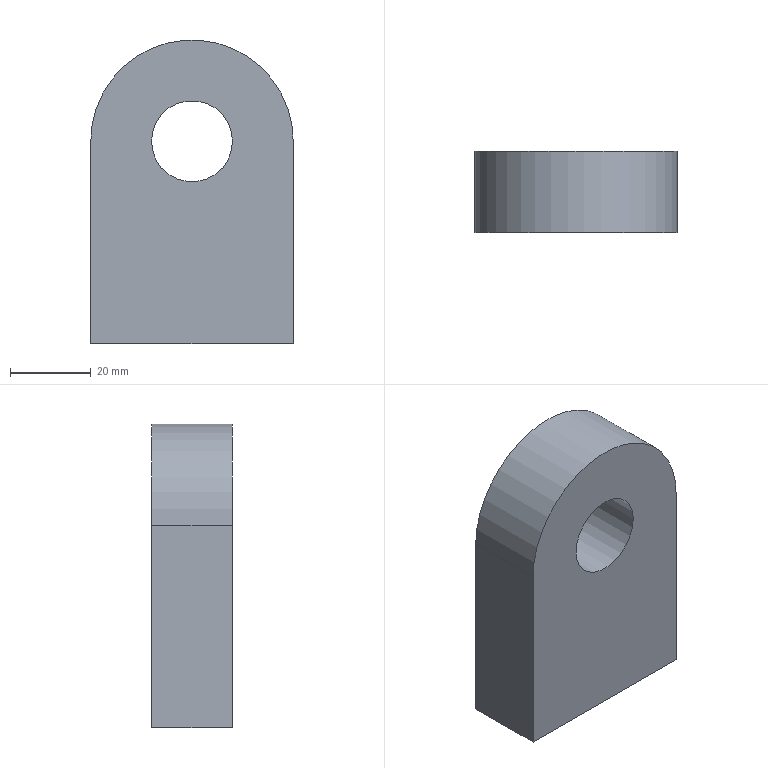Component | NX | BRACKET_1 | 1 solid | 13 faces | box 50 x 20 x 75 mm | volume 62277 mm3 | plane 5 | cylinder 4 | cone 4 | commonest cylinder face diameters 6.8 x2 50 x1 20 x1
STEP:
#1=CARTESIAN_POINT('',(0.,0.,0.));
#2=DIRECTION('',(0.,0.,1.));
#3=DIRECTION('',(1.,0.,0.));
#4=AXIS2_PLACEMENT_3D('',#1,#2,#3);
#5=CARTESIAN_POINT('',(40.5,45.,62.));
#6=VERTEX_POINT('',#5);
#7=CARTESIAN_POINT('',(40.5,45.,12.));
#8=VERTEX_POINT('',#7);
#9=CARTESIAN_POINT('',(40.5,45.,62.));
#10=DIRECTION('',(-0.,0.,-1.));
#11=VECTOR('',#10,1.);
#12=LINE('',#9,#11);
#13=CARTESIAN_POINT('',(40.5,25.,62.));
#14=DIRECTION('',(1.,0.,-0.));
#15=DIRECTION('',(0.,0.,1.));
#16=AXIS2_PLACEMENT_3D('',#13,#14,#15);
#17=PLANE('',#16);
#18=CARTESIAN_POINT('',(0.,-20.));
#19=DIRECTION('',(-1.,0.));
#20=VECTOR('',#19,1.);
#21=LINE('',#18,#20);
#22=(GEOMETRIC_REPRESENTATION_CONTEXT(2)PARAMETRIC_REPRESENTATION_CONTEXT()REPRESENTATION_CONTEXT('',''));
#23=DEFINITIONAL_REPRESENTATION('',(#21),#22);
#24=PCURVE('',#17,#23);
#25=CARTESIAN_POINT('',(65.5,45.,62.));
#26=DIRECTION('',(0.,-1.,0.));
#27=DIRECTION('',(0.,0.,-1.));
#28=AXIS2_PLACEMENT_3D('',#25,#26,#27);
#29=PLANE('',#28);
#30=CARTESIAN_POINT('',(0.,-25.));
#31=DIRECTION('',(1.,-0.));
#32=VECTOR('',#31,1.);
#33=LINE('',#30,#32);
#34=(GEOMETRIC_REPRESENTATION_CONTEXT(2)PARAMETRIC_REPRESENTATION_CONTEXT()REPRESENTATION_CONTEXT('',''));
#35=DEFINITIONAL_REPRESENTATION('',(#33),#34);
#36=PCURVE('',#29,#35);
#37=SURFACE_CURVE('',#12,(#24,#36),.PCURVE_S1.);
#38=EDGE_CURVE('',#6,#8,#37,.T.);
#39=ORIENTED_EDGE('',*,*,#38,.T.);
#40=CARTESIAN_POINT('',(40.5,25.,12.));
#41=VERTEX_POINT('',#40);
#42=CARTESIAN_POINT('',(40.5,25.,12.));
#43=DIRECTION('',(0.,1.,0.));
#44=VECTOR('',#43,1.);
#45=LINE('',#42,#44);
#46=CARTESIAN_POINT('',(-50.,0.));
#47=DIRECTION('',(0.,-1.));
#48=VECTOR('',#47,1.);
#49=LINE('',#46,#48);
#50=(GEOMETRIC_REPRESENTATION_CONTEXT(2)PARAMETRIC_REPRESENTATION_CONTEXT()REPRESENTATION_CONTEXT('',''));
#51=DEFINITIONAL_REPRESENTATION('',(#49),#50);
#52=PCURVE('',#17,#51);
#53=CARTESIAN_POINT('',(40.5,25.,12.));
#54=DIRECTION('',(-0.,0.,1.));
#55=DIRECTION('',(-1.,0.,-0.));
#56=AXIS2_PLACEMENT_3D('',#53,#54,#55);
#57=PLANE('',#56);
#58=CARTESIAN_POINT('',(0.,0.));
#59=DIRECTION('',(0.,-1.));
#60=VECTOR('',#59,1.);
#61=LINE('',#58,#60);
#62=(GEOMETRIC_REPRESENTATION_CONTEXT(2)PARAMETRIC_REPRESENTATION_CONTEXT()REPRESENTATION_CONTEXT('',''));
#63=DEFINITIONAL_REPRESENTATION('',(#61),#62);
#64=PCURVE('',#57,#63);
#65=SURFACE_CURVE('',#45,(#52,#64),.PCURVE_S1.);
#66=EDGE_CURVE('',#41,#8,#65,.T.);
#67=ORIENTED_EDGE('',*,*,#66,.F.);
#68=CARTESIAN_POINT('',(40.5,25.,62.));
#69=VERTEX_POINT('',#68);
#70=CARTESIAN_POINT('',(40.5,25.,62.));
#71=DIRECTION('',(-0.,0.,-1.));
#72=VECTOR('',#71,1.);
#73=LINE('',#70,#72);
#74=CARTESIAN_POINT('',(0.,0.));
#75=DIRECTION('',(-1.,0.));
#76=VECTOR('',#75,1.);
#77=LINE('',#74,#76);
#78=(GEOMETRIC_REPRESENTATION_CONTEXT(2)PARAMETRIC_REPRESENTATION_CONTEXT()REPRESENTATION_CONTEXT('',''));
#79=DEFINITIONAL_REPRESENTATION('',(#77),#78);
#80=PCURVE('',#17,#79);
#81=CARTESIAN_POINT('',(65.5,25.,62.));
#82=DIRECTION('',(0.,-1.,0.));
#83=DIRECTION('',(0.,0.,-1.));
#84=AXIS2_PLACEMENT_3D('',#81,#82,#83);
#85=PLANE('',#84);
#86=CARTESIAN_POINT('',(0.,-25.));
#87=DIRECTION('',(1.,-0.));
#88=VECTOR('',#87,1.);
#89=LINE('',#86,#88);
#90=(GEOMETRIC_REPRESENTATION_CONTEXT(2)PARAMETRIC_REPRESENTATION_CONTEXT()REPRESENTATION_CONTEXT('',''));
#91=DEFINITIONAL_REPRESENTATION('',(#89),#90);
#92=PCURVE('',#85,#91);
#93=SURFACE_CURVE('',#73,(#80,#92),.PCURVE_S1.);
#94=EDGE_CURVE('',#69,#41,#93,.T.);
#95=ORIENTED_EDGE('',*,*,#94,.F.);
#96=CARTESIAN_POINT('',(40.5,25.,62.));
#97=DIRECTION('',(0.,1.,0.));
#98=VECTOR('',#97,1.);
#99=LINE('',#96,#98);
#100=CARTESIAN_POINT('',(0.,0.));
#101=DIRECTION('',(0.,-1.));
#102=VECTOR('',#101,1.);
#103=LINE('',#100,#102);
#104=(GEOMETRIC_REPRESENTATION_CONTEXT(2)PARAMETRIC_REPRESENTATION_CONTEXT()REPRESENTATION_CONTEXT('',''));
#105=DEFINITIONAL_REPRESENTATION('',(#103),#104);
#106=PCURVE('',#17,#105);
#107=CARTESIAN_POINT('',(65.5,25.,62.));
#108=DIRECTION('',(0.,1.,0.));
#109=DIRECTION('',(0.,0.,1.));
#110=AXIS2_PLACEMENT_3D('',#107,#108,#109);
#111=CYLINDRICAL_SURFACE('',#110,25.);
#112=CARTESIAN_POINT('',(-1.571,0.));
#113=DIRECTION('',(0.,1.));
#114=VECTOR('',#113,1.);
#115=LINE('',#112,#114);
#116=(GEOMETRIC_REPRESENTATION_CONTEXT(2)PARAMETRIC_REPRESENTATION_CONTEXT()REPRESENTATION_CONTEXT('',''));
#117=DEFINITIONAL_REPRESENTATION('',(#115),#116);
#118=PCURVE('',#111,#117);
#119=SURFACE_CURVE('',#99,(#106,#118),.PCURVE_S1.);
#120=EDGE_CURVE('',#69,#6,#119,.T.);
#121=ORIENTED_EDGE('',*,*,#120,.T.);
#122=EDGE_LOOP('',(#39,#67,#95,#121));
#123=FACE_BOUND('',#122,.T.);
#124=ADVANCED_FACE('',(#123),#17,.F.);
#125=CARTESIAN_POINT('',(78.5,35.,12.));
#126=VERTEX_POINT('',#125);
#127=CARTESIAN_POINT('',(82.5,35.,12.));
#128=DIRECTION('',(-0.,0.,1.));
#129=DIRECTION('',(-1.,0.,-0.));
#130=AXIS2_PLACEMENT_3D('',#127,#128,#129);
#131=CIRCLE('',#130,4.);
#132=CARTESIAN_POINT('',(-42.,-10.));
#133=DIRECTION('',(1.,0.));
#134=AXIS2_PLACEMENT_2D('',#132,#133);
#135=CIRCLE('',#134,4.);
#136=(GEOMETRIC_REPRESENTATION_CONTEXT(2)PARAMETRIC_REPRESENTATION_CONTEXT()REPRESENTATION_CONTEXT('',''));
#137=DEFINITIONAL_REPRESENTATION('',(#135),#136);
#138=PCURVE('',#57,#137);
#139=CARTESIAN_POINT('',(82.5,35.,12.));
#140=DIRECTION('',(0.,0.,-1.));
#141=DIRECTION('',(0.,1.,0.));
#142=AXIS2_PLACEMENT_3D('',#139,#140,#141);
#143=CONICAL_SURFACE('',#142,4.,0.7854);
#144=CARTESIAN_POINT('',(10.996,0.));
#145=DIRECTION('',(-1.,0.));
#146=VECTOR('',#145,1.);
#147=LINE('',#144,#146);
#148=(GEOMETRIC_REPRESENTATION_CONTEXT(2)PARAMETRIC_REPRESENTATION_CONTEXT()REPRESENTATION_CONTEXT('',''));
#149=DEFINITIONAL_REPRESENTATION('',(#147),#148);
#150=PCURVE('',#143,#149);
#151=SURFACE_CURVE('',#131,(#138,#150),.PCURVE_S1.);
#152=EDGE_CURVE('',#126,#126,#151,.T.);
#153=ORIENTED_EDGE('',*,*,#152,.T.);
#154=EDGE_LOOP('',(#153));
#155=FACE_BOUND('',#154,.T.);
#156=CARTESIAN_POINT('',(44.5,35.,12.));
#157=VERTEX_POINT('',#156);
#158=CARTESIAN_POINT('',(48.5,35.,12.));
#159=DIRECTION('',(-0.,0.,1.));
#160=DIRECTION('',(-1.,0.,-0.));
#161=AXIS2_PLACEMENT_3D('',#158,#159,#160);
#162=CIRCLE('',#161,4.);
#163=CARTESIAN_POINT('',(-8.,-10.));
#164=DIRECTION('',(1.,0.));
#165=AXIS2_PLACEMENT_2D('',#163,#164);
#166=CIRCLE('',#165,4.);
#167=(GEOMETRIC_REPRESENTATION_CONTEXT(2)PARAMETRIC_REPRESENTATION_CONTEXT()REPRESENTATION_CONTEXT('',''));
#168=DEFINITIONAL_REPRESENTATION('',(#166),#167);
#169=PCURVE('',#57,#168);
#170=CARTESIAN_POINT('',(48.5,35.,12.));
#171=DIRECTION('',(0.,0.,-1.));
#172=DIRECTION('',(0.,1.,0.));
#173=AXIS2_PLACEMENT_3D('',#170,#171,#172);
#174=CONICAL_SURFACE('',#173,4.,0.7854);
#175=CARTESIAN_POINT('',(10.996,0.));
#176=DIRECTION('',(-1.,0.));
#177=VECTOR('',#176,1.);
#178=LINE('',#175,#177);
#179=(GEOMETRIC_REPRESENTATION_CONTEXT(2)PARAMETRIC_REPRESENTATION_CONTEXT()REPRESENTATION_CONTEXT('',''));
#180=DEFINITIONAL_REPRESENTATION('',(#178),#179);
#181=PCURVE('',#174,#180);
#182=SURFACE_CURVE('',#162,(#169,#181),.PCURVE_S1.);
#183=EDGE_CURVE('',#157,#157,#182,.T.);
#184=ORIENTED_EDGE('',*,*,#183,.T.);
#185=EDGE_LOOP('',(#184));
#186=FACE_BOUND('',#185,.T.);
#187=CARTESIAN_POINT('',(90.5,45.,12.));
#188=VERTEX_POINT('',#187);
#189=CARTESIAN_POINT('',(40.5,45.,12.));
#190=DIRECTION('',(1.,0.,0.));
#191=VECTOR('',#190,1.);
#192=LINE('',#189,#191);
#193=CARTESIAN_POINT('',(0.,-20.));
#194=DIRECTION('',(-1.,0.));
#195=VECTOR('',#194,1.);
#196=LINE('',#193,#195);
#197=(GEOMETRIC_REPRESENTATION_CONTEXT(2)PARAMETRIC_REPRESENTATION_CONTEXT()REPRESENTATION_CONTEXT('',''));
#198=DEFINITIONAL_REPRESENTATION('',(#196),#197);
#199=PCURVE('',#57,#198);
#200=CARTESIAN_POINT('',(50.,-25.));
#201=DIRECTION('',(-0.,1.));
#202=VECTOR('',#201,1.);
#203=LINE('',#200,#202);
#204=(GEOMETRIC_REPRESENTATION_CONTEXT(2)PARAMETRIC_REPRESENTATION_CONTEXT()REPRESENTATION_CONTEXT('',''));
#205=DEFINITIONAL_REPRESENTATION('',(#203),#204);
#206=PCURVE('',#29,#205);
#207=SURFACE_CURVE('',#192,(#199,#206),.PCURVE_S1.);
#208=EDGE_CURVE('',#8,#188,#207,.T.);
#209=ORIENTED_EDGE('',*,*,#208,.T.);
#210=CARTESIAN_POINT('',(90.5,25.,12.));
#211=VERTEX_POINT('',#210);
#212=CARTESIAN_POINT('',(90.5,25.,12.));
#213=DIRECTION('',(0.,1.,0.));
#214=VECTOR('',#213,1.);
#215=LINE('',#212,#214);
#216=CARTESIAN_POINT('',(-50.,0.));
#217=DIRECTION('',(0.,-1.));
#218=VECTOR('',#217,1.);
#219=LINE('',#216,#218);
#220=(GEOMETRIC_REPRESENTATION_CONTEXT(2)PARAMETRIC_REPRESENTATION_CONTEXT()REPRESENTATION_CONTEXT('',''));
#221=DEFINITIONAL_REPRESENTATION('',(#219),#220);
#222=PCURVE('',#57,#221);
#223=CARTESIAN_POINT('',(90.5,25.,12.));
#224=DIRECTION('',(-1.,0.,-0.));
#225=DIRECTION('',(0.,0.,-1.));
#226=AXIS2_PLACEMENT_3D('',#223,#224,#225);
#227=PLANE('',#226);
#228=CARTESIAN_POINT('',(0.,0.));
#229=DIRECTION('',(0.,-1.));
#230=VECTOR('',#229,1.);
#231=LINE('',#228,#230);
#232=(GEOMETRIC_REPRESENTATION_CONTEXT(2)PARAMETRIC_REPRESENTATION_CONTEXT()REPRESENTATION_CONTEXT('',''));
#233=DEFINITIONAL_REPRESENTATION('',(#231),#232);
#234=PCURVE('',#227,#233);
#235=SURFACE_CURVE('',#215,(#222,#234),.PCURVE_S1.);
#236=EDGE_CURVE('',#211,#188,#235,.T.);
#237=ORIENTED_EDGE('',*,*,#236,.F.);
#238=CARTESIAN_POINT('',(40.5,25.,12.));
#239=DIRECTION('',(1.,0.,0.));
#240=VECTOR('',#239,1.);
#241=LINE('',#238,#240);
#242=CARTESIAN_POINT('',(0.,0.));
#243=DIRECTION('',(-1.,0.));
#244=VECTOR('',#243,1.);
#245=LINE('',#242,#244);
#246=(GEOMETRIC_REPRESENTATION_CONTEXT(2)PARAMETRIC_REPRESENTATION_CONTEXT()REPRESENTATION_CONTEXT('',''));
#247=DEFINITIONAL_REPRESENTATION('',(#245),#246);
#248=PCURVE('',#57,#247);
#249=CARTESIAN_POINT('',(50.,-25.));
#250=DIRECTION('',(-0.,1.));
#251=VECTOR('',#250,1.);
#252=LINE('',#249,#251);
#253=(GEOMETRIC_REPRESENTATION_CONTEXT(2)PARAMETRIC_REPRESENTATION_CONTEXT()REPRESENTATION_CONTEXT('',''));
#254=DEFINITIONAL_REPRESENTATION('',(#252),#253);
#255=PCURVE('',#85,#254);
#256=SURFACE_CURVE('',#241,(#248,#255),.PCURVE_S1.);
#257=EDGE_CURVE('',#41,#211,#256,.T.);
#258=ORIENTED_EDGE('',*,*,#257,.F.);
#259=ORIENTED_EDGE('',*,*,#66,.T.);
#260=EDGE_LOOP('',(#209,#237,#258,#259));
#261=FACE_BOUND('',#260,.T.);
#262=ADVANCED_FACE('',(#155,#186,#261),#57,.F.);
#263=CARTESIAN_POINT('',(90.5,45.,62.));
#264=VERTEX_POINT('',#263);
#265=CARTESIAN_POINT('',(90.5,45.,12.));
#266=DIRECTION('',(-0.,0.,1.));
#267=VECTOR('',#266,1.);
#268=LINE('',#265,#267);
#269=CARTESIAN_POINT('',(0.,-20.));
#270=DIRECTION('',(-1.,0.));
#271=VECTOR('',#270,1.);
#272=LINE('',#269,#271);
#273=(GEOMETRIC_REPRESENTATION_CONTEXT(2)PARAMETRIC_REPRESENTATION_CONTEXT()REPRESENTATION_CONTEXT('',''));
#274=DEFINITIONAL_REPRESENTATION('',(#272),#273);
#275=PCURVE('',#227,#274);
#276=CARTESIAN_POINT('',(50.,25.));
#277=DIRECTION('',(-1.,-0.));
#278=VECTOR('',#277,1.);
#279=LINE('',#276,#278);
#280=(GEOMETRIC_REPRESENTATION_CONTEXT(2)PARAMETRIC_REPRESENTATION_CONTEXT()REPRESENTATION_CONTEXT('',''));
#281=DEFINITIONAL_REPRESENTATION('',(#279),#280);
#282=PCURVE('',#29,#281);
#283=SURFACE_CURVE('',#268,(#275,#282),.PCURVE_S1.);
#284=EDGE_CURVE('',#188,#264,#283,.T.);
#285=ORIENTED_EDGE('',*,*,#284,.T.);
#286=CARTESIAN_POINT('',(90.5,25.,62.));
#287=VERTEX_POINT('',#286);
#288=CARTESIAN_POINT('',(90.5,25.,62.));
#289=DIRECTION('',(0.,1.,0.));
#290=VECTOR('',#289,1.);
#291=LINE('',#288,#290);
#292=CARTESIAN_POINT('',(-50.,0.));
#293=DIRECTION('',(0.,-1.));
#294=VECTOR('',#293,1.);
#295=LINE('',#292,#294);
#296=(GEOMETRIC_REPRESENTATION_CONTEXT(2)PARAMETRIC_REPRESENTATION_CONTEXT()REPRESENTATION_CONTEXT('',''));
#297=DEFINITIONAL_REPRESENTATION('',(#295),#296);
#298=PCURVE('',#227,#297);
#299=CARTESIAN_POINT('',(1.571,0.));
#300=DIRECTION('',(0.,1.));
#301=VECTOR('',#300,1.);
#302=LINE('',#299,#301);
#303=(GEOMETRIC_REPRESENTATION_CONTEXT(2)PARAMETRIC_REPRESENTATION_CONTEXT()REPRESENTATION_CONTEXT('',''));
#304=DEFINITIONAL_REPRESENTATION('',(#302),#303);
#305=PCURVE('',#111,#304);
#306=SURFACE_CURVE('',#291,(#298,#305),.PCURVE_S1.);
#307=EDGE_CURVE('',#287,#264,#306,.T.);
#308=ORIENTED_EDGE('',*,*,#307,.F.);
#309=CARTESIAN_POINT('',(90.5,25.,12.));
#310=DIRECTION('',(-0.,0.,1.));
#311=VECTOR('',#310,1.);
#312=LINE('',#309,#311);
#313=CARTESIAN_POINT('',(0.,0.));
#314=DIRECTION('',(-1.,0.));
#315=VECTOR('',#314,1.);
#316=LINE('',#313,#315);
#317=(GEOMETRIC_REPRESENTATION_CONTEXT(2)PARAMETRIC_REPRESENTATION_CONTEXT()REPRESENTATION_CONTEXT('',''));
#318=DEFINITIONAL_REPRESENTATION('',(#316),#317);
#319=PCURVE('',#227,#318);
#320=CARTESIAN_POINT('',(50.,25.));
#321=DIRECTION('',(-1.,-0.));
#322=VECTOR('',#321,1.);
#323=LINE('',#320,#322);
#324=(GEOMETRIC_REPRESENTATION_CONTEXT(2)PARAMETRIC_REPRESENTATION_CONTEXT()REPRESENTATION_CONTEXT('',''));
#325=DEFINITIONAL_REPRESENTATION('',(#323),#324);
#326=PCURVE('',#85,#325);
#327=SURFACE_CURVE('',#312,(#319,#326),.PCURVE_S1.);
#328=EDGE_CURVE('',#211,#287,#327,.T.);
#329=ORIENTED_EDGE('',*,*,#328,.F.);
#330=ORIENTED_EDGE('',*,*,#236,.T.);
#331=EDGE_LOOP('',(#285,#308,#329,#330));
#332=FACE_BOUND('',#331,.T.);
#333=ADVANCED_FACE('',(#332),#227,.F.);
#334=CARTESIAN_POINT('',(65.5,45.,62.));
#335=DIRECTION('',(0.,-1.,0.));
#336=DIRECTION('',(1.,0.,0.));
#337=AXIS2_PLACEMENT_3D('',#334,#335,#336);
#338=CIRCLE('',#337,25.);
#339=CARTESIAN_POINT('',(1.571,20.));
#340=DIRECTION('',(-1.,0.));
#341=VECTOR('',#340,1.);
#342=LINE('',#339,#341);
#343=(GEOMETRIC_REPRESENTATION_CONTEXT(2)PARAMETRIC_REPRESENTATION_CONTEXT()REPRESENTATION_CONTEXT('',''));
#344=DEFINITIONAL_REPRESENTATION('',(#342),#343);
#345=PCURVE('',#111,#344);
#346=CARTESIAN_POINT('',(0.,0.));
#347=DIRECTION('',(0.,1.));
#348=AXIS2_PLACEMENT_2D('',#346,#347);
#349=CIRCLE('',#348,25.);
#350=(GEOMETRIC_REPRESENTATION_CONTEXT(2)PARAMETRIC_REPRESENTATION_CONTEXT()REPRESENTATION_CONTEXT('',''));
#351=DEFINITIONAL_REPRESENTATION('',(#349),#350);
#352=PCURVE('',#29,#351);
#353=SURFACE_CURVE('',#338,(#345,#352),.PCURVE_S1.);
#354=EDGE_CURVE('',#264,#6,#353,.T.);
#355=ORIENTED_EDGE('',*,*,#354,.T.);
#356=ORIENTED_EDGE('',*,*,#120,.F.);
#357=CARTESIAN_POINT('',(65.5,25.,62.));
#358=DIRECTION('',(0.,-1.,0.));
#359=DIRECTION('',(1.,0.,0.));
#360=AXIS2_PLACEMENT_3D('',#357,#358,#359);
#361=CIRCLE('',#360,25.);
#362=CARTESIAN_POINT('',(1.571,0.));
#363=DIRECTION('',(-1.,0.));
#364=VECTOR('',#363,1.);
#365=LINE('',#362,#364);
#366=(GEOMETRIC_REPRESENTATION_CONTEXT(2)PARAMETRIC_REPRESENTATION_CONTEXT()REPRESENTATION_CONTEXT('',''));
#367=DEFINITIONAL_REPRESENTATION('',(#365),#366);
#368=PCURVE('',#111,#367);
#369=CARTESIAN_POINT('',(0.,0.));
#370=DIRECTION('',(0.,1.));
#371=AXIS2_PLACEMENT_2D('',#369,#370);
#372=CIRCLE('',#371,25.);
#373=(GEOMETRIC_REPRESENTATION_CONTEXT(2)PARAMETRIC_REPRESENTATION_CONTEXT()REPRESENTATION_CONTEXT('',''));
#374=DEFINITIONAL_REPRESENTATION('',(#372),#373);
#375=PCURVE('',#85,#374);
#376=SURFACE_CURVE('',#361,(#368,#375),.PCURVE_S1.);
#377=EDGE_CURVE('',#287,#69,#376,.T.);
#378=ORIENTED_EDGE('',*,*,#377,.F.);
#379=ORIENTED_EDGE('',*,*,#307,.T.);
#380=EDGE_LOOP('',(#355,#356,#378,#379));
#381=FACE_BOUND('',#380,.T.);
#382=ADVANCED_FACE('',(#381),#111,.T.);
#383=CARTESIAN_POINT('',(75.5,25.,62.));
#384=VERTEX_POINT('',#383);
#385=CARTESIAN_POINT('',(65.5,25.,62.));
#386=DIRECTION('',(0.,-1.,0.));
#387=DIRECTION('',(1.,0.,0.));
#388=AXIS2_PLACEMENT_3D('',#385,#386,#387);
#389=CIRCLE('',#388,10.);
#390=CARTESIAN_POINT('',(65.5,25.,62.));
#391=DIRECTION('',(0.,1.,0.));
#392=DIRECTION('',(0.,0.,1.));
#393=AXIS2_PLACEMENT_3D('',#390,#391,#392);
#394=CYLINDRICAL_SURFACE('',#393,10.);
#395=CARTESIAN_POINT('',(7.854,0.));
#396=DIRECTION('',(-1.,0.));
#397=VECTOR('',#396,1.);
#398=LINE('',#395,#397);
#399=(GEOMETRIC_REPRESENTATION_CONTEXT(2)PARAMETRIC_REPRESENTATION_CONTEXT()REPRESENTATION_CONTEXT('',''));
#400=DEFINITIONAL_REPRESENTATION('',(#398),#399);
#401=PCURVE('',#394,#400);
#402=CARTESIAN_POINT('',(0.,0.));
#403=DIRECTION('',(0.,1.));
#404=AXIS2_PLACEMENT_2D('',#402,#403);
#405=CIRCLE('',#404,10.);
#406=(GEOMETRIC_REPRESENTATION_CONTEXT(2)PARAMETRIC_REPRESENTATION_CONTEXT()REPRESENTATION_CONTEXT('',''));
#407=DEFINITIONAL_REPRESENTATION('',(#405),#406);
#408=PCURVE('',#85,#407);
#409=SURFACE_CURVE('',#389,(#401,#408),.PCURVE_S1.);
#410=EDGE_CURVE('',#384,#384,#409,.T.);
#411=ORIENTED_EDGE('',*,*,#410,.F.);
#412=CARTESIAN_POINT('',(75.5,45.,62.));
#413=VERTEX_POINT('',#412);
#414=CARTESIAN_POINT('',(75.5,25.,62.));
#415=CARTESIAN_POINT('',(75.5,45.,62.));
#416=B_SPLINE_CURVE_WITH_KNOTS('',1,(#414,#415),.UNSPECIFIED.,.F.,.F.,(2,2),(0.,20.),.PIECEWISE_BEZIER_KNOTS.);
#417=CARTESIAN_POINT('',(7.854,0.));
#418=DIRECTION('',(0.,1.));
#419=VECTOR('',#418,1.);
#420=LINE('',#417,#419);
#421=(GEOMETRIC_REPRESENTATION_CONTEXT(2)PARAMETRIC_REPRESENTATION_CONTEXT()REPRESENTATION_CONTEXT('',''));
#422=DEFINITIONAL_REPRESENTATION('',(#420),#421);
#423=PCURVE('',#394,#422);
#424=CARTESIAN_POINT('',(1.571,0.));
#425=DIRECTION('',(0.,1.));
#426=VECTOR('',#425,1.);
#427=LINE('',#424,#426);
#428=(GEOMETRIC_REPRESENTATION_CONTEXT(2)PARAMETRIC_REPRESENTATION_CONTEXT()REPRESENTATION_CONTEXT('',''));
#429=DEFINITIONAL_REPRESENTATION('',(#427),#428);
#430=PCURVE('',#394,#429);
#431=SEAM_CURVE('',#416,(#423,#430),.PCURVE_S1.);
#432=EDGE_CURVE('',#384,#413,#431,.T.);
#433=ORIENTED_EDGE('',*,*,#432,.T.);
#434=CARTESIAN_POINT('',(65.5,45.,62.));
#435=DIRECTION('',(0.,-1.,0.));
#436=DIRECTION('',(1.,0.,0.));
#437=AXIS2_PLACEMENT_3D('',#434,#435,#436);
#438=CIRCLE('',#437,10.);
#439=CARTESIAN_POINT('',(7.854,20.));
#440=DIRECTION('',(-1.,0.));
#441=VECTOR('',#440,1.);
#442=LINE('',#439,#441);
#443=(GEOMETRIC_REPRESENTATION_CONTEXT(2)PARAMETRIC_REPRESENTATION_CONTEXT()REPRESENTATION_CONTEXT('',''));
#444=DEFINITIONAL_REPRESENTATION('',(#442),#443);
#445=PCURVE('',#394,#444);
#446=CARTESIAN_POINT('',(0.,0.));
#447=DIRECTION('',(0.,1.));
#448=AXIS2_PLACEMENT_2D('',#446,#447);
#449=CIRCLE('',#448,10.);
#450=(GEOMETRIC_REPRESENTATION_CONTEXT(2)PARAMETRIC_REPRESENTATION_CONTEXT()REPRESENTATION_CONTEXT('',''));
#451=DEFINITIONAL_REPRESENTATION('',(#449),#450);
#452=PCURVE('',#29,#451);
#453=SURFACE_CURVE('',#438,(#445,#452),.PCURVE_S1.);
#454=EDGE_CURVE('',#413,#413,#453,.T.);
#455=ORIENTED_EDGE('',*,*,#454,.T.);
#456=ORIENTED_EDGE('',*,*,#432,.F.);
#457=EDGE_LOOP('',(#411,#433,#455,#456));
#458=FACE_BOUND('',#457,.F.);
#459=ADVANCED_FACE('',(#458),#394,.F.);
#460=ORIENTED_EDGE('',*,*,#94,.T.);
#461=ORIENTED_EDGE('',*,*,#257,.T.);
#462=ORIENTED_EDGE('',*,*,#328,.T.);
#463=ORIENTED_EDGE('',*,*,#377,.T.);
#464=EDGE_LOOP('',(#460,#461,#462,#463));
#465=FACE_BOUND('',#464,.T.);
#466=ORIENTED_EDGE('',*,*,#410,.F.);
#467=EDGE_LOOP('',(#466));
#468=FACE_BOUND('',#467,.T.);
#469=ADVANCED_FACE('',(#465,#468),#85,.T.);
#470=ORIENTED_EDGE('',*,*,#38,.F.);
#471=ORIENTED_EDGE('',*,*,#354,.F.);
#472=ORIENTED_EDGE('',*,*,#284,.F.);
#473=ORIENTED_EDGE('',*,*,#208,.F.);
#474=EDGE_LOOP('',(#470,#471,#472,#473));
#475=FACE_BOUND('',#474,.T.);
#476=ORIENTED_EDGE('',*,*,#454,.T.);
#477=EDGE_LOOP('',(#476));
#478=FACE_BOUND('',#477,.T.);
#479=ADVANCED_FACE('',(#475,#478),#29,.F.);
#480=CARTESIAN_POINT('',(51.9,35.,26.));
#481=VERTEX_POINT('',#480);
#482=CARTESIAN_POINT('',(45.1,35.,26.));
#483=VERTEX_POINT('',#482);
#484=CARTESIAN_POINT('',(48.5,35.,26.));
#485=DIRECTION('',(0.,0.,-1.));
#486=DIRECTION('',(-1.,0.,-0.));
#487=AXIS2_PLACEMENT_3D('',#484,#485,#486);
#488=CIRCLE('',#487,3.4);
#489=CARTESIAN_POINT('',(48.5,35.,26.));
#490=DIRECTION('',(0.,0.,-1.));
#491=DIRECTION('',(1.,0.,0.));
#492=AXIS2_PLACEMENT_3D('',#489,#490,#491);
#493=CONICAL_SURFACE('',#492,3.4,1.03);
#494=CARTESIAN_POINT('',(-3.142,-0.));
#495=DIRECTION('',(1.,0.));
#496=VECTOR('',#495,1.);
#497=LINE('',#494,#496);
#498=(GEOMETRIC_REPRESENTATION_CONTEXT(2)PARAMETRIC_REPRESENTATION_CONTEXT()REPRESENTATION_CONTEXT('',''));
#499=DEFINITIONAL_REPRESENTATION('',(#497),#498);
#500=PCURVE('',#493,#499);
#501=CARTESIAN_POINT('',(48.5,35.,12.));
#502=DIRECTION('',(-0.,0.,1.));
#503=DIRECTION('',(-1.,0.,-0.));
#504=AXIS2_PLACEMENT_3D('',#501,#502,#503);
#505=CYLINDRICAL_SURFACE('',#504,3.4);
#506=CARTESIAN_POINT('',(6.283,14.));
#507=DIRECTION('',(-1.,0.));
#508=VECTOR('',#507,1.);
#509=LINE('',#506,#508);
#510=(GEOMETRIC_REPRESENTATION_CONTEXT(2)PARAMETRIC_REPRESENTATION_CONTEXT()REPRESENTATION_CONTEXT('',''));
#511=DEFINITIONAL_REPRESENTATION('',(#509),#510);
#512=PCURVE('',#505,#511);
#513=SURFACE_CURVE('',#488,(#500,#512),.PCURVE_S1.);
#514=EDGE_CURVE('',#481,#483,#513,.T.);
#515=ORIENTED_EDGE('',*,*,#514,.F.);
#516=CARTESIAN_POINT('',(48.5,35.,28.043));
#517=VERTEX_POINT('',#516);
#518=CARTESIAN_POINT('',(48.5,35.,28.043));
#519=CARTESIAN_POINT('',(51.9,35.,26.));
#520=B_SPLINE_CURVE_WITH_KNOTS('',1,(#518,#519),.UNSPECIFIED.,.F.,.F.,(2,2),(-3.967,-0.),.PIECEWISE_BEZIER_KNOTS.);
#521=CARTESIAN_POINT('',(0.,0.));
#522=DIRECTION('',(0.,1.));
#523=VECTOR('',#522,1.);
#524=LINE('',#521,#523);
#525=(GEOMETRIC_REPRESENTATION_CONTEXT(2)PARAMETRIC_REPRESENTATION_CONTEXT()REPRESENTATION_CONTEXT('',''));
#526=DEFINITIONAL_REPRESENTATION('',(#524),#525);
#527=PCURVE('',#493,#526);
#528=CARTESIAN_POINT('',(6.283,0.));
#529=DIRECTION('',(0.,1.));
#530=VECTOR('',#529,1.);
#531=LINE('',#528,#530);
#532=(GEOMETRIC_REPRESENTATION_CONTEXT(2)PARAMETRIC_REPRESENTATION_CONTEXT()REPRESENTATION_CONTEXT('',''));
#533=DEFINITIONAL_REPRESENTATION('',(#531),#532);
#534=PCURVE('',#493,#533);
#535=SEAM_CURVE('',#520,(#527,#534),.PCURVE_S1.);
#536=EDGE_CURVE('',#517,#481,#535,.T.);
#537=ORIENTED_EDGE('',*,*,#536,.F.);
#538=ORIENTED_EDGE('',*,*,#536,.T.);
#539=CARTESIAN_POINT('',(48.5,35.,26.));
#540=DIRECTION('',(0.,0.,-1.));
#541=DIRECTION('',(-1.,0.,-0.));
#542=AXIS2_PLACEMENT_3D('',#539,#540,#541);
#543=CIRCLE('',#542,3.4);
#544=CARTESIAN_POINT('',(3.142,-0.));
#545=DIRECTION('',(1.,0.));
#546=VECTOR('',#545,1.);
#547=LINE('',#544,#546);
#548=(GEOMETRIC_REPRESENTATION_CONTEXT(2)PARAMETRIC_REPRESENTATION_CONTEXT()REPRESENTATION_CONTEXT('',''));
#549=DEFINITIONAL_REPRESENTATION('',(#547),#548);
#550=PCURVE('',#493,#549);
#551=CARTESIAN_POINT('',(6.283,14.));
#552=DIRECTION('',(-1.,0.));
#553=VECTOR('',#552,1.);
#554=LINE('',#551,#553);
#555=(GEOMETRIC_REPRESENTATION_CONTEXT(2)PARAMETRIC_REPRESENTATION_CONTEXT()REPRESENTATION_CONTEXT('',''));
#556=DEFINITIONAL_REPRESENTATION('',(#554),#555);
#557=PCURVE('',#505,#556);
#558=SURFACE_CURVE('',#543,(#550,#557),.PCURVE_S1.);
#559=EDGE_CURVE('',#483,#481,#558,.T.);
#560=ORIENTED_EDGE('',*,*,#559,.F.);
#561=EDGE_LOOP('',(#515,#537,#538,#560));
#562=FACE_BOUND('',#561,.F.);
#563=ADVANCED_FACE('',(#562),#493,.F.);
#564=CARTESIAN_POINT('',(45.1,35.,12.6));
#565=VERTEX_POINT('',#564);
#566=CARTESIAN_POINT('',(48.5,31.6,12.6));
#567=VERTEX_POINT('',#566);
#568=CARTESIAN_POINT('',(48.5,35.,12.6));
#569=DIRECTION('',(0.,0.,-1.));
#570=DIRECTION('',(0.,-1.,0.));
#571=AXIS2_PLACEMENT_3D('',#568,#569,#570);
#572=CIRCLE('',#571,3.4);
#573=CARTESIAN_POINT('',(7.854,0.6));
#574=DIRECTION('',(-1.,0.));
#575=VECTOR('',#574,1.);
#576=LINE('',#573,#575);
#577=(GEOMETRIC_REPRESENTATION_CONTEXT(2)PARAMETRIC_REPRESENTATION_CONTEXT()REPRESENTATION_CONTEXT('',''));
#578=DEFINITIONAL_REPRESENTATION('',(#576),#577);
#579=PCURVE('',#505,#578);
#580=CARTESIAN_POINT('',(3.142,-0.6));
#581=DIRECTION('',(1.,0.));
#582=VECTOR('',#581,1.);
#583=LINE('',#580,#582);
#584=(GEOMETRIC_REPRESENTATION_CONTEXT(2)PARAMETRIC_REPRESENTATION_CONTEXT()REPRESENTATION_CONTEXT('',''));
#585=DEFINITIONAL_REPRESENTATION('',(#583),#584);
#586=PCURVE('',#174,#585);
#587=SURFACE_CURVE('',#572,(#579,#586),.PCURVE_S1.);
#588=EDGE_CURVE('',#565,#567,#587,.T.);
#589=ORIENTED_EDGE('',*,*,#588,.F.);
#590=CARTESIAN_POINT('',(45.1,35.,12.6));
#591=CARTESIAN_POINT('',(45.1,35.,26.));
#592=B_SPLINE_CURVE_WITH_KNOTS('',1,(#590,#591),.UNSPECIFIED.,.F.,.F.,(2,2),(0.6,14.),.PIECEWISE_BEZIER_KNOTS.);
#593=CARTESIAN_POINT('',(6.283,0.));
#594=DIRECTION('',(0.,1.));
#595=VECTOR('',#594,1.);
#596=LINE('',#593,#595);
#597=(GEOMETRIC_REPRESENTATION_CONTEXT(2)PARAMETRIC_REPRESENTATION_CONTEXT()REPRESENTATION_CONTEXT('',''));
#598=DEFINITIONAL_REPRESENTATION('',(#596),#597);
#599=PCURVE('',#505,#598);
#600=CARTESIAN_POINT('',(0.,0.));
#601=DIRECTION('',(0.,1.));
#602=VECTOR('',#601,1.);
#603=LINE('',#600,#602);
#604=(GEOMETRIC_REPRESENTATION_CONTEXT(2)PARAMETRIC_REPRESENTATION_CONTEXT()REPRESENTATION_CONTEXT('',''));
#605=DEFINITIONAL_REPRESENTATION('',(#603),#604);
#606=PCURVE('',#505,#605);
#607=SEAM_CURVE('',#592,(#599,#606),.PCURVE_S1.);
#608=EDGE_CURVE('',#565,#483,#607,.T.);
#609=ORIENTED_EDGE('',*,*,#608,.T.);
#610=ORIENTED_EDGE('',*,*,#559,.T.);
#611=ORIENTED_EDGE('',*,*,#514,.T.);
#612=ORIENTED_EDGE('',*,*,#608,.F.);
#613=CARTESIAN_POINT('',(48.5,35.,12.6));
#614=DIRECTION('',(0.,0.,-1.));
#615=DIRECTION('',(0.,-1.,0.));
#616=AXIS2_PLACEMENT_3D('',#613,#614,#615);
#617=CIRCLE('',#616,3.4);
#618=CARTESIAN_POINT('',(1.571,0.6));
#619=DIRECTION('',(-1.,0.));
#620=VECTOR('',#619,1.);
#621=LINE('',#618,#620);
#622=(GEOMETRIC_REPRESENTATION_CONTEXT(2)PARAMETRIC_REPRESENTATION_CONTEXT()REPRESENTATION_CONTEXT('',''));
#623=DEFINITIONAL_REPRESENTATION('',(#621),#622);
#624=PCURVE('',#505,#623);
#625=CARTESIAN_POINT('',(9.425,-0.6));
#626=DIRECTION('',(1.,0.));
#627=VECTOR('',#626,1.);
#628=LINE('',#625,#627);
#629=(GEOMETRIC_REPRESENTATION_CONTEXT(2)PARAMETRIC_REPRESENTATION_CONTEXT()REPRESENTATION_CONTEXT('',''));
#630=DEFINITIONAL_REPRESENTATION('',(#628),#629);
#631=PCURVE('',#174,#630);
#632=SURFACE_CURVE('',#617,(#624,#631),.PCURVE_S1.);
#633=EDGE_CURVE('',#567,#565,#632,.T.);
#634=ORIENTED_EDGE('',*,*,#633,.F.);
#635=EDGE_LOOP('',(#589,#609,#610,#611,#612,#634));
#636=FACE_BOUND('',#635,.F.);
#637=ADVANCED_FACE('',(#636),#505,.F.);
#638=ORIENTED_EDGE('',*,*,#588,.T.);
#639=ORIENTED_EDGE('',*,*,#633,.T.);
#640=CARTESIAN_POINT('',(45.1,35.,12.6));
#641=CARTESIAN_POINT('',(44.5,35.,12.));
#642=B_SPLINE_CURVE_WITH_KNOTS('',1,(#640,#641),.UNSPECIFIED.,.F.,.F.,(2,2),(-0.8485,0.),.PIECEWISE_BEZIER_KNOTS.);
#643=CARTESIAN_POINT('',(10.996,0.));
#644=DIRECTION('',(0.,1.));
#645=VECTOR('',#644,1.);
#646=LINE('',#643,#645);
#647=(GEOMETRIC_REPRESENTATION_CONTEXT(2)PARAMETRIC_REPRESENTATION_CONTEXT()REPRESENTATION_CONTEXT('',''));
#648=DEFINITIONAL_REPRESENTATION('',(#646),#647);
#649=PCURVE('',#174,#648);
#650=CARTESIAN_POINT('',(4.712,0.));
#651=DIRECTION('',(0.,1.));
#652=VECTOR('',#651,1.);
#653=LINE('',#650,#652);
#654=(GEOMETRIC_REPRESENTATION_CONTEXT(2)PARAMETRIC_REPRESENTATION_CONTEXT()REPRESENTATION_CONTEXT('',''));
#655=DEFINITIONAL_REPRESENTATION('',(#653),#654);
#656=PCURVE('',#174,#655);
#657=SEAM_CURVE('',#642,(#649,#656),.PCURVE_S1.);
#658=EDGE_CURVE('',#565,#157,#657,.T.);
#659=ORIENTED_EDGE('',*,*,#658,.T.);
#660=ORIENTED_EDGE('',*,*,#183,.T.);
#661=ORIENTED_EDGE('',*,*,#658,.F.);
#662=EDGE_LOOP('',(#638,#639,#659,#660,#661));
#663=FACE_BOUND('',#662,.F.);
#664=ADVANCED_FACE('',(#663),#174,.F.);
#665=CARTESIAN_POINT('',(85.9,35.,26.));
#666=VERTEX_POINT('',#665);
#667=CARTESIAN_POINT('',(79.1,35.,26.));
#668=VERTEX_POINT('',#667);
#669=CARTESIAN_POINT('',(82.5,35.,26.));
#670=DIRECTION('',(0.,0.,-1.));
#671=DIRECTION('',(-1.,0.,-0.));
#672=AXIS2_PLACEMENT_3D('',#669,#670,#671);
#673=CIRCLE('',#672,3.4);
#674=CARTESIAN_POINT('',(82.5,35.,26.));
#675=DIRECTION('',(0.,0.,-1.));
#676=DIRECTION('',(1.,0.,0.));
#677=AXIS2_PLACEMENT_3D('',#674,#675,#676);
#678=CONICAL_SURFACE('',#677,3.4,1.03);
#679=CARTESIAN_POINT('',(-3.142,0.));
#680=DIRECTION('',(1.,0.));
#681=VECTOR('',#680,1.);
#682=LINE('',#679,#681);
#683=(GEOMETRIC_REPRESENTATION_CONTEXT(2)PARAMETRIC_REPRESENTATION_CONTEXT()REPRESENTATION_CONTEXT('',''));
#684=DEFINITIONAL_REPRESENTATION('',(#682),#683);
#685=PCURVE('',#678,#684);
#686=CARTESIAN_POINT('',(82.5,35.,12.));
#687=DIRECTION('',(-0.,0.,1.));
#688=DIRECTION('',(-1.,0.,-0.));
#689=AXIS2_PLACEMENT_3D('',#686,#687,#688);
#690=CYLINDRICAL_SURFACE('',#689,3.4);
#691=CARTESIAN_POINT('',(6.283,14.));
#692=DIRECTION('',(-1.,0.));
#693=VECTOR('',#692,1.);
#694=LINE('',#691,#693);
#695=(GEOMETRIC_REPRESENTATION_CONTEXT(2)PARAMETRIC_REPRESENTATION_CONTEXT()REPRESENTATION_CONTEXT('',''));
#696=DEFINITIONAL_REPRESENTATION('',(#694),#695);
#697=PCURVE('',#690,#696);
#698=SURFACE_CURVE('',#673,(#685,#697),.PCURVE_S1.);
#699=EDGE_CURVE('',#666,#668,#698,.T.);
#700=ORIENTED_EDGE('',*,*,#699,.F.);
#701=CARTESIAN_POINT('',(82.5,35.,28.043));
#702=VERTEX_POINT('',#701);
#703=CARTESIAN_POINT('',(82.5,35.,28.043));
#704=CARTESIAN_POINT('',(85.9,35.,26.));
#705=B_SPLINE_CURVE_WITH_KNOTS('',1,(#703,#704),.UNSPECIFIED.,.F.,.F.,(2,2),(-3.967,0.),.PIECEWISE_BEZIER_KNOTS.);
#706=CARTESIAN_POINT('',(0.,0.));
#707=DIRECTION('',(0.,1.));
#708=VECTOR('',#707,1.);
#709=LINE('',#706,#708);
#710=(GEOMETRIC_REPRESENTATION_CONTEXT(2)PARAMETRIC_REPRESENTATION_CONTEXT()REPRESENTATION_CONTEXT('',''));
#711=DEFINITIONAL_REPRESENTATION('',(#709),#710);
#712=PCURVE('',#678,#711);
#713=CARTESIAN_POINT('',(6.283,0.));
#714=DIRECTION('',(0.,1.));
#715=VECTOR('',#714,1.);
#716=LINE('',#713,#715);
#717=(GEOMETRIC_REPRESENTATION_CONTEXT(2)PARAMETRIC_REPRESENTATION_CONTEXT()REPRESENTATION_CONTEXT('',''));
#718=DEFINITIONAL_REPRESENTATION('',(#716),#717);
#719=PCURVE('',#678,#718);
#720=SEAM_CURVE('',#705,(#712,#719),.PCURVE_S1.);
#721=EDGE_CURVE('',#702,#666,#720,.T.);
#722=ORIENTED_EDGE('',*,*,#721,.F.);
#723=ORIENTED_EDGE('',*,*,#721,.T.);
#724=CARTESIAN_POINT('',(82.5,35.,26.));
#725=DIRECTION('',(0.,0.,-1.));
#726=DIRECTION('',(-1.,0.,-0.));
#727=AXIS2_PLACEMENT_3D('',#724,#725,#726);
#728=CIRCLE('',#727,3.4);
#729=CARTESIAN_POINT('',(3.142,0.));
#730=DIRECTION('',(1.,0.));
#731=VECTOR('',#730,1.);
#732=LINE('',#729,#731);
#733=(GEOMETRIC_REPRESENTATION_CONTEXT(2)PARAMETRIC_REPRESENTATION_CONTEXT()REPRESENTATION_CONTEXT('',''));
#734=DEFINITIONAL_REPRESENTATION('',(#732),#733);
#735=PCURVE('',#678,#734);
#736=CARTESIAN_POINT('',(6.283,14.));
#737=DIRECTION('',(-1.,0.));
#738=VECTOR('',#737,1.);
#739=LINE('',#736,#738);
#740=(GEOMETRIC_REPRESENTATION_CONTEXT(2)PARAMETRIC_REPRESENTATION_CONTEXT()REPRESENTATION_CONTEXT('',''));
#741=DEFINITIONAL_REPRESENTATION('',(#739),#740);
#742=PCURVE('',#690,#741);
#743=SURFACE_CURVE('',#728,(#735,#742),.PCURVE_S1.);
#744=EDGE_CURVE('',#668,#666,#743,.T.);
#745=ORIENTED_EDGE('',*,*,#744,.F.);
#746=EDGE_LOOP('',(#700,#722,#723,#745));
#747=FACE_BOUND('',#746,.F.);
#748=ADVANCED_FACE('',(#747),#678,.F.);
#749=CARTESIAN_POINT('',(79.1,35.,12.6));
#750=VERTEX_POINT('',#749);
#751=CARTESIAN_POINT('',(82.5,31.6,12.6));
#752=VERTEX_POINT('',#751);
#753=CARTESIAN_POINT('',(82.5,35.,12.6));
#754=DIRECTION('',(0.,0.,-1.));
#755=DIRECTION('',(0.,-1.,0.));
#756=AXIS2_PLACEMENT_3D('',#753,#754,#755);
#757=CIRCLE('',#756,3.4);
#758=CARTESIAN_POINT('',(7.854,0.6));
#759=DIRECTION('',(-1.,0.));
#760=VECTOR('',#759,1.);
#761=LINE('',#758,#760);
#762=(GEOMETRIC_REPRESENTATION_CONTEXT(2)PARAMETRIC_REPRESENTATION_CONTEXT()REPRESENTATION_CONTEXT('',''));
#763=DEFINITIONAL_REPRESENTATION('',(#761),#762);
#764=PCURVE('',#690,#763);
#765=CARTESIAN_POINT('',(3.142,-0.6));
#766=DIRECTION('',(1.,-0.));
#767=VECTOR('',#766,1.);
#768=LINE('',#765,#767);
#769=(GEOMETRIC_REPRESENTATION_CONTEXT(2)PARAMETRIC_REPRESENTATION_CONTEXT()REPRESENTATION_CONTEXT('',''));
#770=DEFINITIONAL_REPRESENTATION('',(#768),#769);
#771=PCURVE('',#143,#770);
#772=SURFACE_CURVE('',#757,(#764,#771),.PCURVE_S1.);
#773=EDGE_CURVE('',#750,#752,#772,.T.);
#774=ORIENTED_EDGE('',*,*,#773,.F.);
#775=CARTESIAN_POINT('',(79.1,35.,12.6));
#776=CARTESIAN_POINT('',(79.1,35.,26.));
#777=B_SPLINE_CURVE_WITH_KNOTS('',1,(#775,#776),.UNSPECIFIED.,.F.,.F.,(2,2),(0.6,14.),.PIECEWISE_BEZIER_KNOTS.);
#778=CARTESIAN_POINT('',(6.283,0.));
#779=DIRECTION('',(0.,1.));
#780=VECTOR('',#779,1.);
#781=LINE('',#778,#780);
#782=(GEOMETRIC_REPRESENTATION_CONTEXT(2)PARAMETRIC_REPRESENTATION_CONTEXT()REPRESENTATION_CONTEXT('',''));
#783=DEFINITIONAL_REPRESENTATION('',(#781),#782);
#784=PCURVE('',#690,#783);
#785=CARTESIAN_POINT('',(0.,0.));
#786=DIRECTION('',(0.,1.));
#787=VECTOR('',#786,1.);
#788=LINE('',#785,#787);
#789=(GEOMETRIC_REPRESENTATION_CONTEXT(2)PARAMETRIC_REPRESENTATION_CONTEXT()REPRESENTATION_CONTEXT('',''));
#790=DEFINITIONAL_REPRESENTATION('',(#788),#789);
#791=PCURVE('',#690,#790);
#792=SEAM_CURVE('',#777,(#784,#791),.PCURVE_S1.);
#793=EDGE_CURVE('',#750,#668,#792,.T.);
#794=ORIENTED_EDGE('',*,*,#793,.T.);
#795=ORIENTED_EDGE('',*,*,#744,.T.);
#796=ORIENTED_EDGE('',*,*,#699,.T.);
#797=ORIENTED_EDGE('',*,*,#793,.F.);
#798=CARTESIAN_POINT('',(82.5,35.,12.6));
#799=DIRECTION('',(0.,0.,-1.));
#800=DIRECTION('',(0.,-1.,0.));
#801=AXIS2_PLACEMENT_3D('',#798,#799,#800);
#802=CIRCLE('',#801,3.4);
#803=CARTESIAN_POINT('',(1.571,0.6));
#804=DIRECTION('',(-1.,0.));
#805=VECTOR('',#804,1.);
#806=LINE('',#803,#805);
#807=(GEOMETRIC_REPRESENTATION_CONTEXT(2)PARAMETRIC_REPRESENTATION_CONTEXT()REPRESENTATION_CONTEXT('',''));
#808=DEFINITIONAL_REPRESENTATION('',(#806),#807);
#809=PCURVE('',#690,#808);
#810=CARTESIAN_POINT('',(9.425,-0.6));
#811=DIRECTION('',(1.,0.));
#812=VECTOR('',#811,1.);
#813=LINE('',#810,#812);
#814=(GEOMETRIC_REPRESENTATION_CONTEXT(2)PARAMETRIC_REPRESENTATION_CONTEXT()REPRESENTATION_CONTEXT('',''));
#815=DEFINITIONAL_REPRESENTATION('',(#813),#814);
#816=PCURVE('',#143,#815);
#817=SURFACE_CURVE('',#802,(#809,#816),.PCURVE_S1.);
#818=EDGE_CURVE('',#752,#750,#817,.T.);
#819=ORIENTED_EDGE('',*,*,#818,.F.);
#820=EDGE_LOOP('',(#774,#794,#795,#796,#797,#819));
#821=FACE_BOUND('',#820,.F.);
#822=ADVANCED_FACE('',(#821),#690,.F.);
#823=ORIENTED_EDGE('',*,*,#773,.T.);
#824=ORIENTED_EDGE('',*,*,#818,.T.);
#825=CARTESIAN_POINT('',(79.1,35.,12.6));
#826=CARTESIAN_POINT('',(78.5,35.,12.));
#827=B_SPLINE_CURVE_WITH_KNOTS('',1,(#825,#826),.UNSPECIFIED.,.F.,.F.,(2,2),(-0.8485,0.),.PIECEWISE_BEZIER_KNOTS.);
#828=CARTESIAN_POINT('',(10.996,0.));
#829=DIRECTION('',(0.,1.));
#830=VECTOR('',#829,1.);
#831=LINE('',#828,#830);
#832=(GEOMETRIC_REPRESENTATION_CONTEXT(2)PARAMETRIC_REPRESENTATION_CONTEXT()REPRESENTATION_CONTEXT('',''));
#833=DEFINITIONAL_REPRESENTATION('',(#831),#832);
#834=PCURVE('',#143,#833);
#835=CARTESIAN_POINT('',(4.712,0.));
#836=DIRECTION('',(0.,1.));
#837=VECTOR('',#836,1.);
#838=LINE('',#835,#837);
#839=(GEOMETRIC_REPRESENTATION_CONTEXT(2)PARAMETRIC_REPRESENTATION_CONTEXT()REPRESENTATION_CONTEXT('',''));
#840=DEFINITIONAL_REPRESENTATION('',(#838),#839);
#841=PCURVE('',#143,#840);
#842=SEAM_CURVE('',#827,(#834,#841),.PCURVE_S1.);
#843=EDGE_CURVE('',#750,#126,#842,.T.);
#844=ORIENTED_EDGE('',*,*,#843,.T.);
#845=ORIENTED_EDGE('',*,*,#152,.T.);
#846=ORIENTED_EDGE('',*,*,#843,.F.);
#847=EDGE_LOOP('',(#823,#824,#844,#845,#846));
#848=FACE_BOUND('',#847,.F.);
#849=ADVANCED_FACE('',(#848),#143,.F.);
#850=CLOSED_SHELL('',(#124,#262,#333,#382,#459,#469,#479,#563,#637,#664,#748,#822,#849));
#851=MANIFOLD_SOLID_BREP('',#850);
#852=(LENGTH_UNIT()NAMED_UNIT(*)SI_UNIT(.MILLI.,.METRE.));
#853=UNCERTAINTY_MEASURE_WITH_UNIT(LENGTH_MEASURE(0.000005),#852,'','');
#854=(NAMED_UNIT(*)PLANE_ANGLE_UNIT()SI_UNIT($,.RADIAN.));
#855=(NAMED_UNIT(*)SI_UNIT($,.STERADIAN.)SOLID_ANGLE_UNIT());
#856=(GEOMETRIC_REPRESENTATION_CONTEXT(3)GLOBAL_UNCERTAINTY_ASSIGNED_CONTEXT((#853))GLOBAL_UNIT_ASSIGNED_CONTEXT((#852,#854,#855))REPRESENTATION_CONTEXT('',''));
#857=ADVANCED_BREP_SHAPE_REPRESENTATION('',(#4,#851),#856);